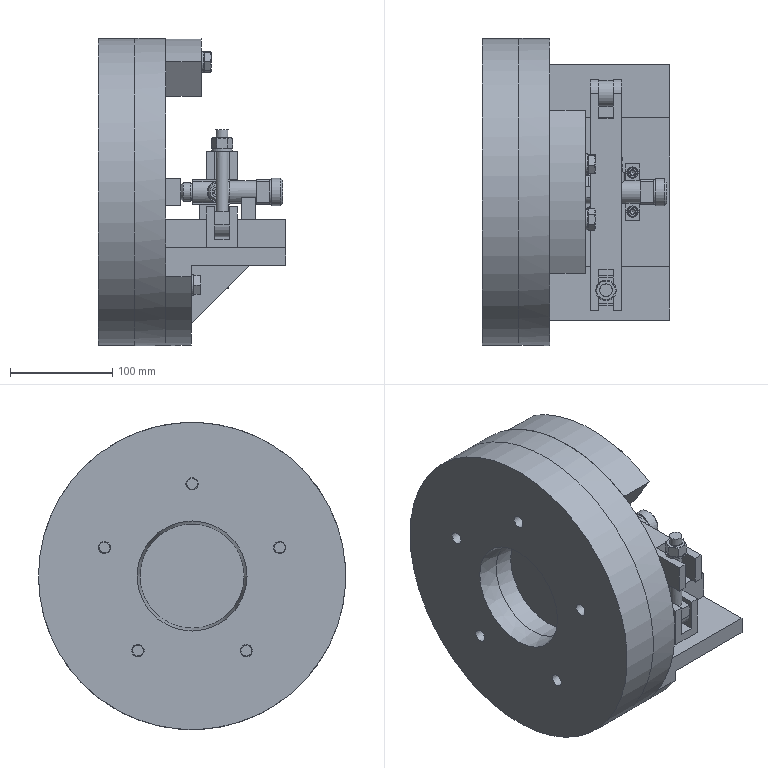Assembly | NX | mm | 45 component files | 45 solids | 870 faces | box 183.5 x 300 x 300 mm | volume 6122971 mm3 | plane 460 | cone 200 | cylinder 178 | torus 31 | sphere 1 | commonest cylinder face diameters 12 x23 6 x22 20 x17 10 x13 18 x10 11.701 x9 6.6 x8 11 x8
Bill of materials:
GB-T70.1-2000,M6x25 | 2 |  | Hexagon Socket Head Cap Screw, GB-T 70.1-2000,M6x25
unnamed part 1 | 1 |  | Obround (stadium-shaped) thick plate with two through holes, one near each rounded end.
GB-T848-2002,M12 | 6 |  | Flat annular ring (plain washer-like disc): a thin circular plate with a single concentric through-hole, flat parallel faces and straight cylindrical inner and outer edges.
GB-T119.1-2000,12x30 | 1 |  | Parallel Pin, GB-T 119.1-2000,12x30
unnamed part 2 | 1 |  | Curved annular-sector block (arc segment) with a concentric arc-shaped through slot with rounded ends.
unnamed part 3 | 1 |  | Slender cylindrical rod with an eye at one end: a short cylindrical boss with a transverse through hole, and a shaft with stepped/reduced-diameter sections along its length.
GB-T70.1-2000,M6x16 | 6 |  | Hexagon Socket Head Cap Screw, GB-T 70.1-2000,M6x16
GB-T5782-2000,M12x50 | 2 |  | Hexagon Head Bolt, GB-T 5782-2000,M12x50
unnamed part 4 | 1 |  | Long rectangular bar with open-ended slots cut into both ends forming forked ends; one end is rounded with a transverse through hole across the fork, the other end is square.
unnamed part 5 | 2 |  | Rectangular block with four through holes in its largest face, arranged in two pairs near each end; two holes appear larger than the other two.
GB-T6170_F-2000,M12x1.75 | 3 |  | Hexagonal nut-shaped body with central round bore, chamfered hex corners on both faces and a chamfer/countersink at the bore edge.
unnamed part 6 | 1 |  | Flat circular disc/flange with a large central bore, a thin raised annular step around the bore on one face, and five small through holes on a bolt circle.
GB-T5782-2000,M12x40 | 2 |  | Hexagon Head Bolt, GB-T 5782-2000,M12x40
GB-T119.1-2000,8x30 | 1 |  | Parallel Pin, GB-T 119.1-2000,8x30
unnamed part 7 | 1 |  | Rectangular block with a central V-shaped notch with a flat-bottomed narrow slot at its base, and a vertical through hole in each raised end section.
GB-T70.1-2000,M12x40 | 5 |  | Hexagon Socket Head Cap Screw, GB-T 70.1-2000,M12x40
GB-T119.1-2000,6x26 | 4 |  | Parallel Pin, GB-T 119.1-2000,6x26
unnamed part 8 | 1 |  | Thick circular plate with multiple holes: five larger through holes on a circle, four smaller chamfered/countersunk-looking holes near the rim, two tiny holes near the center, and a narrow radial slot or step cut in from the edge.
unnamed part 9 | 1 |  | Multi-port tubular fitting body: a main cylindrical run with ports at both ends and two perpendicular side branches offset along the axis, with stepped/grooved barb-like ends, wrench-type flats, and a circular recess with small hole on one face.
unnamed part 10 | 1 |  | Clevis/fork-shaped block: rectangular U-shaped body with two parallel prongs, a transverse through hole across both prongs, and a short cylindrical stub projecting from the base.
unnamed part 11 | 1 |  | Eye-end rod: a block head with one rounded end and a transverse through hole, with a long cylindrical shaft rising from the flat side and a reduced-diameter groove near the shaft tip.
unnamed part 12 | 1 |  | Elongated rectangular block-like part with a raised central pad between two lower end flanges. Each flange has one larger round hole. The raised top face has a small cluster of small holes. In one view the underside has a curved, circular-segment profile.
Mates:
1. concentric | fixture_body 1 edge | adapter_plate 1 edge
2. concentric | angle_bar 1 edge | fixture_body 1 edge
3. touch align | fixed_v_block 1 face | angle_bar 1 face
4. center | fixed_v_block 1 face | fixed_v_block 1 face | angle_bar 1 face | angle_bar 1 face
5. distance | four_way_valve_body 1 face | fixed_v_block 1 face
6. distance | four_way_valve_body 1 face | angle_bar 1 face
7. fix | adapter_plate 1 component
8. touch align | fixture_body 1 face | adapter_plate 1 face
9. touch align | parallel_ref_block 2 face | angle_bar 1 face
10. center | parallel_ref_block 2 face | parallel_ref_block 2 face | angle_bar 1 face | angle_bar 1 face
11. distance | parallel_ref_block 2 face | fixed_v_block 1 face
12. touch align | four_way_valve_body 1 face | fixture_body 1 face
13. touch align | parallel_ref_block 1 face | fixture_body 1 face
14. center | parallel_ref_block 1 face | parallel_ref_block 1 face | angle_bar 1 face | angle_bar 1 face
15. distance | parallel_ref_block 1 face | angle_bar 1 face
16. concentric | slider 1 edge | angle_bar 1 arc
17. concentric | hinge_link 1 edge | angle_bar 1 arc
18. concentric | hinge_screw 1 edge | hinge_link 1 edge
19. touch align | fixed_screw 1 face | angle_bar 1 face
20. touch align | clamp_plate 1 face | four_way_valve_body 1 face
21. parallel | clamp_plate 1 face | angle_bar 1 face
22. fix | angle_bar 1 component
23. concentric | fixed_screw 1 edge | clamp_plate 1 edge
24. concentric | counterweight_block 1 edge | fixture_body 1 edge
25. bond | fixture_body 1 component | assembly component
26. bond | GB-T70_1-2000_M12x40 5 component | assembly component
27. bond | GB-T70_1-2000_M12x40 4 component | assembly component
28. circular | assembly datumaxis | assembly cartesiancoordinatesystem | assembly cartesiancoordinatesystem | assembly cartesiancoordinatesystem | assembly cartesiancoordinatesystem | assembly cartesiancoordinatesystem
29. bond | GB-T70_1-2000_M12x40 3 component | assembly component
30. bond | GB-T70_1-2000_M12x40 2 component | assembly component
31. bond | GB-T70_1-2000_M12x40 1 component | assembly component
32. concentric | GB-T848-2002_M12 6 edge | GB-T5782-2000_M12x40 2 edge
33. touch align | GB-T848-2002_M12 6 face | angle_bar 1 face
34. touch align | GB-T5782-2000_M12x40 2 face | fixture_body 1 face
35. bond | angle_bar 1 component | assembly component
36. bond | GB-T5782-2000_M12x40 2 component | assembly component
37. bond | GB-T848-2002_M12 6 component | assembly component
38. bond | GB-T5782-2000_M12x40 1 component | assembly component
39. bond | GB-T848-2002_M12 5 component | assembly component
40. linear | assembly datumaxis | assembly cartesiancoordinatesystem | assembly cartesiancoordinatesystem
41. linear | assembly datumaxis | assembly cartesiancoordinatesystem | assembly cartesiancoordinatesystem
42. concentric | GB-T848-2002_M12 4 edge | GB-T5782-2000_M12x50 2 edge
43. touch align | GB-T848-2002_M12 4 face | counterweight_block 1 face
44. touch align | GB-T5782-2000_M12x50 2 face | fixture_body 1 face
45. bond | counterweight_block 1 component | assembly component
46. bond | GB-T5782-2000_M12x50 2 component | assembly component
47. bond | GB-T848-2002_M12 4 component | assembly component
48. bond | GB-T5782-2000_M12x50 1 component | assembly component
49. bond | GB-T848-2002_M12 3 component | assembly component
50. circular | assembly datumaxis | assembly cartesiancoordinatesystem | assembly cartesiancoordinatesystem
51. circular | assembly datumaxis | assembly cartesiancoordinatesystem | assembly cartesiancoordinatesystem
52. concentric | GB-T848-2002_M12 2 edge | GB-T6170_F-2000_M12x1_75 3 edge
53. touch align | GB-T848-2002_M12 2 face | hinge_screw 1 face
54. touch align | GB-T848-2002_M12 2 face | clamp_plate 1 face
55. concentric | GB-T6170_F-2000_M12x1_75 2 edge | angle_bar 1 arc
56. concentric | GB-T848-2002_M12 1 edge | angle_bar 1 arc
57. concentric | GB-T6170_F-2000_M12x1_75 1 edge | GB-T848-2002_M12 1 edge